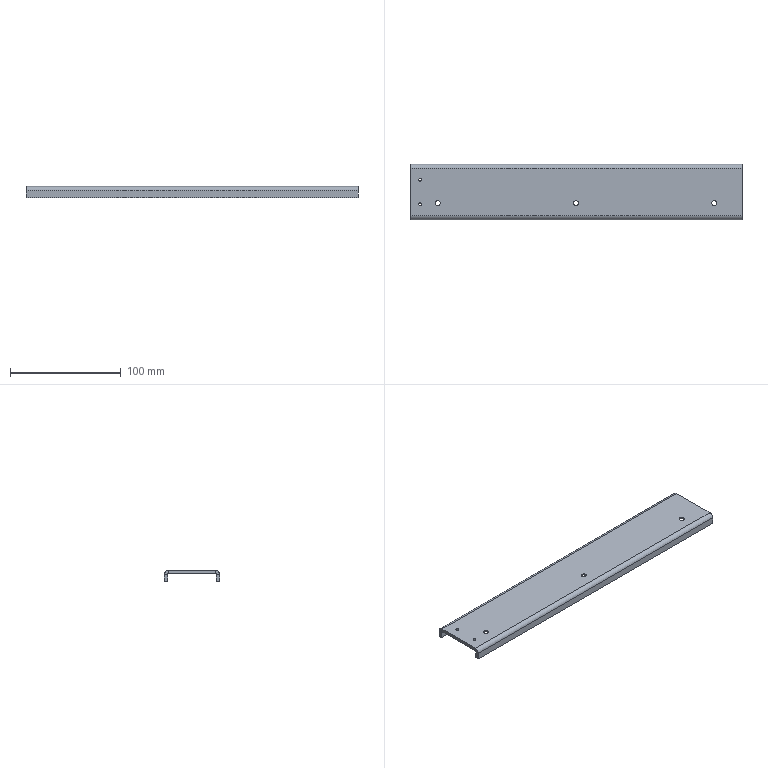Component | SolidWorks | SFTJ-04-DragChainSheet-Metal-1 | 1 solid | 38 faces | box 300 x 50 x 10 mm | volume 55526 mm3 | plane 18 | cylinder 14 | cone 6 | commonest cylinder face diameters 4.5 x6 2.5 x4 7.473 x2 1.473 x2 | material 201 Annealed Stainless Steel (SS)
STEP:
#1=COLOUR_RGB('',0.7922,0.8196,0.9333);
#2=FILL_AREA_STYLE_COLOUR('',#1);
#3=FILL_AREA_STYLE('',(#2));
#4=SURFACE_STYLE_FILL_AREA(#3);
#5=SURFACE_SIDE_STYLE('',(#4));
#6=SURFACE_STYLE_USAGE(.BOTH.,#5);
#7=PRESENTATION_STYLE_ASSIGNMENT((#6));
#8=CARTESIAN_POINT('',(-6.557,-0.5228,-1.827));
#9=VERTEX_POINT('',#8);
#10=CARTESIAN_POINT('',(-6.656,-0.5228,-1.827));
#11=VERTEX_POINT('',#10);
#12=CARTESIAN_POINT('',(-6.607,-0.5228,-1.827));
#13=DIRECTION('',(0.,-0.,-1.));
#14=DIRECTION('',(-1.,0.,0.));
#15=AXIS2_PLACEMENT_3D('',#12,#13,#14);
#16=CIRCLE('',#15,0.04921);
#17=EDGE_CURVE('',#9,#11,#16,.T.);
#18=ORIENTED_EDGE('',*,*,#17,.F.);
#19=CARTESIAN_POINT('',(-6.557,-0.5228,-1.945));
#20=VERTEX_POINT('',#19);
#21=CARTESIAN_POINT('',(-6.557,-0.5228,-1.945));
#22=DIRECTION('',(0.,-0.,-1.));
#23=VECTOR('',#22,39.37);
#24=LINE('',#21,#23);
#25=EDGE_CURVE('',#9,#20,#24,.T.);
#26=ORIENTED_EDGE('',*,*,#25,.T.);
#27=CARTESIAN_POINT('',(-6.656,-0.5228,-1.945));
#28=VERTEX_POINT('',#27);
#29=CARTESIAN_POINT('',(-6.607,-0.5228,-1.945));
#30=DIRECTION('',(0.,-0.,-1.));
#31=DIRECTION('',(-1.,0.,0.));
#32=AXIS2_PLACEMENT_3D('',#29,#30,#31);
#33=CIRCLE('',#32,0.04921);
#34=EDGE_CURVE('',#20,#28,#33,.T.);
#35=ORIENTED_EDGE('',*,*,#34,.T.);
#36=CARTESIAN_POINT('',(-6.656,-0.5228,-1.945));
#37=DIRECTION('',(0.,-0.,-1.));
#38=VECTOR('',#37,39.37);
#39=LINE('',#36,#38);
#40=EDGE_CURVE('',#11,#28,#39,.T.);
#41=ORIENTED_EDGE('',*,*,#40,.F.);
#42=EDGE_LOOP('',(#18,#26,#35,#41));
#43=FACE_OUTER_BOUND('',#42,.T.);
#44=CARTESIAN_POINT('',(-6.607,-0.5228,-1.945));
#45=DIRECTION('',(0.,-0.,-1.));
#46=DIRECTION('',(-1.,0.,0.));
#47=AXIS2_PLACEMENT_3D('',#44,#45,#46);
#48=CYLINDRICAL_SURFACE('',#47,0.04921);
#49=ADVANCED_FACE('',(#43),#48,.F.);
#50=CARTESIAN_POINT('',(-6.557,0.3433,-1.827));
#51=VERTEX_POINT('',#50);
#52=CARTESIAN_POINT('',(-6.656,0.3433,-1.827));
#53=VERTEX_POINT('',#52);
#54=CARTESIAN_POINT('',(-6.607,0.3433,-1.827));
#55=DIRECTION('',(0.,-0.,-1.));
#56=DIRECTION('',(-1.,0.,0.));
#57=AXIS2_PLACEMENT_3D('',#54,#55,#56);
#58=CIRCLE('',#57,0.04921);
#59=EDGE_CURVE('',#51,#53,#58,.T.);
#60=ORIENTED_EDGE('',*,*,#59,.F.);
#61=CARTESIAN_POINT('',(-6.557,0.3433,-1.945));
#62=VERTEX_POINT('',#61);
#63=CARTESIAN_POINT('',(-6.557,0.3433,-1.945));
#64=DIRECTION('',(0.,-0.,-1.));
#65=VECTOR('',#64,39.37);
#66=LINE('',#63,#65);
#67=EDGE_CURVE('',#51,#62,#66,.T.);
#68=ORIENTED_EDGE('',*,*,#67,.T.);
#69=CARTESIAN_POINT('',(-6.656,0.3433,-1.945));
#70=VERTEX_POINT('',#69);
#71=CARTESIAN_POINT('',(-6.607,0.3433,-1.945));
#72=DIRECTION('',(0.,-0.,-1.));
#73=DIRECTION('',(-1.,0.,0.));
#74=AXIS2_PLACEMENT_3D('',#71,#72,#73);
#75=CIRCLE('',#74,0.04921);
#76=EDGE_CURVE('',#62,#70,#75,.T.);
#77=ORIENTED_EDGE('',*,*,#76,.T.);
#78=CARTESIAN_POINT('',(-6.656,0.3433,-1.945));
#79=DIRECTION('',(0.,-0.,-1.));
#80=VECTOR('',#79,39.37);
#81=LINE('',#78,#80);
#82=EDGE_CURVE('',#53,#70,#81,.T.);
#83=ORIENTED_EDGE('',*,*,#82,.F.);
#84=EDGE_LOOP('',(#60,#68,#77,#83));
#85=FACE_OUTER_BOUND('',#84,.T.);
#86=CARTESIAN_POINT('',(-6.607,0.3433,-1.945));
#87=DIRECTION('',(0.,-0.,-1.));
#88=DIRECTION('',(-1.,0.,0.));
#89=AXIS2_PLACEMENT_3D('',#86,#87,#88);
#90=CYLINDRICAL_SURFACE('',#89,0.04921);
#91=ADVANCED_FACE('',(#85),#90,.F.);
#92=CARTESIAN_POINT('',(-5.896,-0.4834,-1.849));
#93=VERTEX_POINT('',#92);
#94=CARTESIAN_POINT('',(-6.073,-0.4834,-1.849));
#95=VERTEX_POINT('',#94);
#96=CARTESIAN_POINT('',(-5.985,-0.4834,-1.849));
#97=DIRECTION('',(0.,-0.,-1.));
#98=DIRECTION('',(-1.,0.,0.));
#99=AXIS2_PLACEMENT_3D('',#96,#97,#98);
#100=CIRCLE('',#99,0.08858);
#101=EDGE_CURVE('',#93,#95,#100,.T.);
#102=ORIENTED_EDGE('',*,*,#101,.F.);
#103=CARTESIAN_POINT('',(-5.8,-0.4834,-1.945));
#104=VERTEX_POINT('',#103);
#105=CARTESIAN_POINT('',(-5.8,-0.4834,-1.945));
#106=DIRECTION('',(0.7071,-0.,-0.7071));
#107=VECTOR('',#106,39.37);
#108=LINE('',#105,#107);
#109=EDGE_CURVE('',#93,#104,#108,.T.);
#110=ORIENTED_EDGE('',*,*,#109,.T.);
#111=CARTESIAN_POINT('',(-6.17,-0.4834,-1.945));
#112=VERTEX_POINT('',#111);
#113=CARTESIAN_POINT('',(-5.985,-0.4834,-1.945));
#114=DIRECTION('',(0.,-0.,-1.));
#115=DIRECTION('',(-1.,0.,0.));
#116=AXIS2_PLACEMENT_3D('',#113,#114,#115);
#117=CIRCLE('',#116,0.185);
#118=EDGE_CURVE('',#104,#112,#117,.T.);
#119=ORIENTED_EDGE('',*,*,#118,.T.);
#120=CARTESIAN_POINT('',(-6.17,-0.4834,-1.945));
#121=DIRECTION('',(-0.7071,-0.,-0.7071));
#122=VECTOR('',#121,39.37);
#123=LINE('',#120,#122);
#124=EDGE_CURVE('',#95,#112,#123,.T.);
#125=ORIENTED_EDGE('',*,*,#124,.F.);
#126=EDGE_LOOP('',(#102,#110,#119,#125));
#127=FACE_OUTER_BOUND('',#126,.T.);
#128=CARTESIAN_POINT('',(-5.985,-0.4834,-1.945));
#129=DIRECTION('',(0.,-0.,-1.));
#130=DIRECTION('',(-1.,0.,0.));
#131=AXIS2_PLACEMENT_3D('',#128,#129,#130);
#132=CONICAL_SURFACE('',#131,0.185,0.7854);
#133=ADVANCED_FACE('',(#127),#132,.F.);
#134=CARTESIAN_POINT('',(-5.896,-0.4834,-1.827));
#135=VERTEX_POINT('',#134);
#136=CARTESIAN_POINT('',(-6.073,-0.4834,-1.827));
#137=VERTEX_POINT('',#136);
#138=CARTESIAN_POINT('',(-5.985,-0.4834,-1.827));
#139=DIRECTION('',(0.,-0.,-1.));
#140=DIRECTION('',(-1.,0.,0.));
#141=AXIS2_PLACEMENT_3D('',#138,#139,#140);
#142=CIRCLE('',#141,0.08858);
#143=EDGE_CURVE('',#135,#137,#142,.T.);
#144=ORIENTED_EDGE('',*,*,#143,.F.);
#145=CARTESIAN_POINT('',(-5.896,-0.4834,-1.945));
#146=DIRECTION('',(0.,-0.,-1.));
#147=VECTOR('',#146,39.37);
#148=LINE('',#145,#147);
#149=EDGE_CURVE('',#135,#93,#148,.T.);
#150=ORIENTED_EDGE('',*,*,#149,.T.);
#151=ORIENTED_EDGE('',*,*,#101,.T.);
#152=CARTESIAN_POINT('',(-6.073,-0.4834,-1.945));
#153=DIRECTION('',(0.,-0.,-1.));
#154=VECTOR('',#153,39.37);
#155=LINE('',#152,#154);
#156=EDGE_CURVE('',#137,#95,#155,.T.);
#157=ORIENTED_EDGE('',*,*,#156,.F.);
#158=EDGE_LOOP('',(#144,#150,#151,#157));
#159=FACE_OUTER_BOUND('',#158,.T.);
#160=CARTESIAN_POINT('',(-5.985,-0.4834,-1.945));
#161=DIRECTION('',(0.,-0.,-1.));
#162=DIRECTION('',(-1.,0.,0.));
#163=AXIS2_PLACEMENT_3D('',#160,#161,#162);
#164=CYLINDRICAL_SURFACE('',#163,0.08858);
#165=ADVANCED_FACE('',(#159),#164,.F.);
#166=CARTESIAN_POINT('',(-0.9748,-0.4834,-1.849));
#167=VERTEX_POINT('',#166);
#168=CARTESIAN_POINT('',(-1.152,-0.4834,-1.849));
#169=VERTEX_POINT('',#168);
#170=CARTESIAN_POINT('',(-1.063,-0.4834,-1.849));
#171=DIRECTION('',(0.,-0.,-1.));
#172=DIRECTION('',(-1.,0.,0.));
#173=AXIS2_PLACEMENT_3D('',#170,#171,#172);
#174=CIRCLE('',#173,0.08858);
#175=EDGE_CURVE('',#167,#169,#174,.T.);
#176=ORIENTED_EDGE('',*,*,#175,.F.);
#177=CARTESIAN_POINT('',(-0.8783,-0.4834,-1.945));
#178=VERTEX_POINT('',#177);
#179=CARTESIAN_POINT('',(-0.8783,-0.4834,-1.945));
#180=DIRECTION('',(0.7071,-0.,-0.7071));
#181=VECTOR('',#180,39.37);
#182=LINE('',#179,#181);
#183=EDGE_CURVE('',#167,#178,#182,.T.);
#184=ORIENTED_EDGE('',*,*,#183,.T.);
#185=CARTESIAN_POINT('',(-1.248,-0.4834,-1.945));
#186=VERTEX_POINT('',#185);
#187=CARTESIAN_POINT('',(-1.063,-0.4834,-1.945));
#188=DIRECTION('',(0.,-0.,-1.));
#189=DIRECTION('',(-1.,0.,0.));
#190=AXIS2_PLACEMENT_3D('',#187,#188,#189);
#191=CIRCLE('',#190,0.185);
#192=EDGE_CURVE('',#178,#186,#191,.T.);
#193=ORIENTED_EDGE('',*,*,#192,.T.);
#194=CARTESIAN_POINT('',(-1.248,-0.4834,-1.945));
#195=DIRECTION('',(-0.7071,-0.,-0.7071));
#196=VECTOR('',#195,39.37);
#197=LINE('',#194,#196);
#198=EDGE_CURVE('',#169,#186,#197,.T.);
#199=ORIENTED_EDGE('',*,*,#198,.F.);
#200=EDGE_LOOP('',(#176,#184,#193,#199));
#201=FACE_OUTER_BOUND('',#200,.T.);
#202=CARTESIAN_POINT('',(-1.063,-0.4834,-1.945));
#203=DIRECTION('',(0.,-0.,-1.));
#204=DIRECTION('',(-1.,0.,0.));
#205=AXIS2_PLACEMENT_3D('',#202,#203,#204);
#206=CONICAL_SURFACE('',#205,0.185,0.7854);
#207=ADVANCED_FACE('',(#201),#206,.F.);
#208=CARTESIAN_POINT('',(-0.9748,-0.4834,-1.827));
#209=VERTEX_POINT('',#208);
#210=CARTESIAN_POINT('',(-1.152,-0.4834,-1.827));
#211=VERTEX_POINT('',#210);
#212=CARTESIAN_POINT('',(-1.063,-0.4834,-1.827));
#213=DIRECTION('',(0.,-0.,-1.));
#214=DIRECTION('',(-1.,0.,0.));
#215=AXIS2_PLACEMENT_3D('',#212,#213,#214);
#216=CIRCLE('',#215,0.08858);
#217=EDGE_CURVE('',#209,#211,#216,.T.);
#218=ORIENTED_EDGE('',*,*,#217,.F.);
#219=CARTESIAN_POINT('',(-0.9748,-0.4834,-1.945));
#220=DIRECTION('',(0.,-0.,-1.));
#221=VECTOR('',#220,39.37);
#222=LINE('',#219,#221);
#223=EDGE_CURVE('',#209,#167,#222,.T.);
#224=ORIENTED_EDGE('',*,*,#223,.T.);
#225=ORIENTED_EDGE('',*,*,#175,.T.);
#226=CARTESIAN_POINT('',(-1.152,-0.4834,-1.945));
#227=DIRECTION('',(0.,-0.,-1.));
#228=VECTOR('',#227,39.37);
#229=LINE('',#226,#228);
#230=EDGE_CURVE('',#211,#169,#229,.T.);
#231=ORIENTED_EDGE('',*,*,#230,.F.);
#232=EDGE_LOOP('',(#218,#224,#225,#231));
#233=FACE_OUTER_BOUND('',#232,.T.);
#234=CARTESIAN_POINT('',(-1.063,-0.4834,-1.945));
#235=DIRECTION('',(0.,-0.,-1.));
#236=DIRECTION('',(-1.,0.,0.));
#237=AXIS2_PLACEMENT_3D('',#234,#235,#236);
#238=CYLINDRICAL_SURFACE('',#237,0.08858);
#239=ADVANCED_FACE('',(#233),#238,.F.);
#240=CARTESIAN_POINT('',(3.946,-0.4834,-1.849));
#241=VERTEX_POINT('',#240);
#242=CARTESIAN_POINT('',(3.769,-0.4834,-1.849));
#243=VERTEX_POINT('',#242);
#244=CARTESIAN_POINT('',(3.858,-0.4834,-1.849));
#245=DIRECTION('',(0.,-0.,-1.));
#246=DIRECTION('',(-1.,0.,0.));
#247=AXIS2_PLACEMENT_3D('',#244,#245,#246);
#248=CIRCLE('',#247,0.08858);
#249=EDGE_CURVE('',#241,#243,#248,.T.);
#250=ORIENTED_EDGE('',*,*,#249,.F.);
#251=CARTESIAN_POINT('',(4.043,-0.4834,-1.945));
#252=VERTEX_POINT('',#251);
#253=CARTESIAN_POINT('',(4.043,-0.4834,-1.945));
#254=DIRECTION('',(0.7071,-0.,-0.7071));
#255=VECTOR('',#254,39.37);
#256=LINE('',#253,#255);
#257=EDGE_CURVE('',#241,#252,#256,.T.);
#258=ORIENTED_EDGE('',*,*,#257,.T.);
#259=CARTESIAN_POINT('',(3.673,-0.4834,-1.945));
#260=VERTEX_POINT('',#259);
#261=CARTESIAN_POINT('',(3.858,-0.4834,-1.945));
#262=DIRECTION('',(0.,-0.,-1.));
#263=DIRECTION('',(-1.,0.,0.));
#264=AXIS2_PLACEMENT_3D('',#261,#262,#263);
#265=CIRCLE('',#264,0.185);
#266=EDGE_CURVE('',#252,#260,#265,.T.);
#267=ORIENTED_EDGE('',*,*,#266,.T.);
#268=CARTESIAN_POINT('',(3.673,-0.4834,-1.945));
#269=DIRECTION('',(-0.7071,-0.,-0.7071));
#270=VECTOR('',#269,39.37);
#271=LINE('',#268,#270);
#272=EDGE_CURVE('',#243,#260,#271,.T.);
#273=ORIENTED_EDGE('',*,*,#272,.F.);
#274=EDGE_LOOP('',(#250,#258,#267,#273));
#275=FACE_OUTER_BOUND('',#274,.T.);
#276=CARTESIAN_POINT('',(3.858,-0.4834,-1.945));
#277=DIRECTION('',(0.,-0.,-1.));
#278=DIRECTION('',(-1.,0.,0.));
#279=AXIS2_PLACEMENT_3D('',#276,#277,#278);
#280=CONICAL_SURFACE('',#279,0.185,0.7854);
#281=ADVANCED_FACE('',(#275),#280,.F.);
#282=CARTESIAN_POINT('',(3.946,-0.4834,-1.827));
#283=VERTEX_POINT('',#282);
#284=CARTESIAN_POINT('',(3.769,-0.4834,-1.827));
#285=VERTEX_POINT('',#284);
#286=CARTESIAN_POINT('',(3.858,-0.4834,-1.827));
#287=DIRECTION('',(0.,-0.,-1.));
#288=DIRECTION('',(-1.,0.,0.));
#289=AXIS2_PLACEMENT_3D('',#286,#287,#288);
#290=CIRCLE('',#289,0.08858);
#291=EDGE_CURVE('',#283,#285,#290,.T.);
#292=ORIENTED_EDGE('',*,*,#291,.F.);
#293=CARTESIAN_POINT('',(3.946,-0.4834,-1.945));
#294=DIRECTION('',(0.,-0.,-1.));
#295=VECTOR('',#294,39.37);
#296=LINE('',#293,#295);
#297=EDGE_CURVE('',#283,#241,#296,.T.);
#298=ORIENTED_EDGE('',*,*,#297,.T.);
#299=ORIENTED_EDGE('',*,*,#249,.T.);
#300=CARTESIAN_POINT('',(3.769,-0.4834,-1.945));
#301=DIRECTION('',(0.,-0.,-1.));
#302=VECTOR('',#301,39.37);
#303=LINE('',#300,#302);
#304=EDGE_CURVE('',#285,#243,#303,.T.);
#305=ORIENTED_EDGE('',*,*,#304,.F.);
#306=EDGE_LOOP('',(#292,#298,#299,#305));
#307=FACE_OUTER_BOUND('',#306,.T.);
#308=CARTESIAN_POINT('',(3.858,-0.4834,-1.945));
#309=DIRECTION('',(0.,-0.,-1.));
#310=DIRECTION('',(-1.,0.,0.));
#311=AXIS2_PLACEMENT_3D('',#308,#309,#310);
#312=CYLINDRICAL_SURFACE('',#311,0.08858);
#313=ADVANCED_FACE('',(#307),#312,.F.);
#314=CARTESIAN_POINT('',(-6.969,0.7474,-1.827));
#315=VERTEX_POINT('',#314);
#316=CARTESIAN_POINT('',(-6.969,0.7474,-1.945));
#317=VERTEX_POINT('',#316);
#318=CARTESIAN_POINT('',(-6.969,0.7474,-1.827));
#319=DIRECTION('',(0.,-0.,-1.));
#320=VECTOR('',#319,39.37);
#321=LINE('',#318,#320);
#322=EDGE_CURVE('',#315,#317,#321,.T.);
#323=ORIENTED_EDGE('',*,*,#322,.F.);
#324=CARTESIAN_POINT('',(-6.969,0.8945,-1.974));
#325=VERTEX_POINT('',#324);
#326=CARTESIAN_POINT('',(-6.969,0.7474,-1.974));
#327=DIRECTION('',(1.,0.,0.));
#328=DIRECTION('',(0.,1.,0.));
#329=AXIS2_PLACEMENT_3D('',#326,#327,#328);
#330=CIRCLE('',#329,0.1471);
#331=EDGE_CURVE('',#325,#315,#330,.T.);
#332=ORIENTED_EDGE('',*,*,#331,.F.);
#333=CARTESIAN_POINT('',(-6.969,0.7764,-1.974));
#334=VERTEX_POINT('',#333);
#335=CARTESIAN_POINT('',(-6.969,0.7764,-1.974));
#336=DIRECTION('',(0.,1.,-0.));
#337=VECTOR('',#336,39.37);
#338=LINE('',#335,#337);
#339=EDGE_CURVE('',#334,#325,#338,.T.);
#340=ORIENTED_EDGE('',*,*,#339,.F.);
#341=CARTESIAN_POINT('',(-6.969,0.7474,-1.974));
#342=DIRECTION('',(1.,0.,0.));
#343=DIRECTION('',(0.,1.,0.));
#344=AXIS2_PLACEMENT_3D('',#341,#342,#343);
#345=CIRCLE('',#344,0.029);
#346=EDGE_CURVE('',#334,#317,#345,.T.);
#347=ORIENTED_EDGE('',*,*,#346,.T.);
#348=EDGE_LOOP('',(#323,#332,#340,#347));
#349=FACE_OUTER_BOUND('',#348,.T.);
#350=CARTESIAN_POINT('',(-6.969,0.7474,-1.827));
#351=DIRECTION('',(-1.,-0.,-0.));
#352=DIRECTION('',(0.,1.,-0.));
#353=AXIS2_PLACEMENT_3D('',#350,#351,#352);
#354=PLANE('',#353);
#355=ADVANCED_FACE('',(#349),#354,.T.);
#356=CARTESIAN_POINT('',(-6.969,-0.9269,-1.827));
#357=VERTEX_POINT('',#356);
#358=CARTESIAN_POINT('',(-6.969,-1.074,-1.827));
#359=DIRECTION('',(0.,-1.,0.));
#360=VECTOR('',#359,39.37);
#361=LINE('',#358,#360);
#362=EDGE_CURVE('',#315,#357,#361,.T.);
#363=ORIENTED_EDGE('',*,*,#362,.F.);
#364=ORIENTED_EDGE('',*,*,#322,.T.);
#365=CARTESIAN_POINT('',(-6.969,-0.9269,-1.945));
#366=VERTEX_POINT('',#365);
#367=CARTESIAN_POINT('',(-6.969,-1.074,-1.945));
#368=DIRECTION('',(0.,-1.,0.));
#369=VECTOR('',#368,39.37);
#370=LINE('',#367,#369);
#371=EDGE_CURVE('',#317,#366,#370,.T.);
#372=ORIENTED_EDGE('',*,*,#371,.T.);
#373=CARTESIAN_POINT('',(-6.969,-0.9269,-1.945));
#374=DIRECTION('',(-0.,0.,1.));
#375=VECTOR('',#374,39.37);
#376=LINE('',#373,#375);
#377=EDGE_CURVE('',#366,#357,#376,.T.);
#378=ORIENTED_EDGE('',*,*,#377,.T.);
#379=EDGE_LOOP('',(#363,#364,#372,#378));
#380=FACE_OUTER_BOUND('',#379,.T.);
#381=CARTESIAN_POINT('',(-6.969,0.7764,-1.974));
#382=DIRECTION('',(-1.,-0.,-0.));
#383=DIRECTION('',(0.,1.,-0.));
#384=AXIS2_PLACEMENT_3D('',#381,#382,#383);
#385=PLANE('',#384);
#386=ADVANCED_FACE('',(#380),#385,.T.);
#387=CARTESIAN_POINT('',(4.842,0.8945,-1.974));
#388=VERTEX_POINT('',#387);
#389=CARTESIAN_POINT('',(4.842,0.7764,-1.974));
#390=VERTEX_POINT('',#389);
#391=CARTESIAN_POINT('',(4.842,0.8945,-1.974));
#392=DIRECTION('',(0.,-1.,0.));
#393=VECTOR('',#392,39.37);
#394=LINE('',#391,#393);
#395=EDGE_CURVE('',#388,#390,#394,.T.);
#396=ORIENTED_EDGE('',*,*,#395,.F.);
#397=CARTESIAN_POINT('',(4.842,0.7474,-1.827));
#398=VERTEX_POINT('',#397);
#399=CARTESIAN_POINT('',(4.842,0.7474,-1.974));
#400=DIRECTION('',(1.,0.,0.));
#401=DIRECTION('',(0.,1.,0.));
#402=AXIS2_PLACEMENT_3D('',#399,#400,#401);
#403=CIRCLE('',#402,0.1471);
#404=EDGE_CURVE('',#388,#398,#403,.T.);
#405=ORIENTED_EDGE('',*,*,#404,.T.);
#406=CARTESIAN_POINT('',(4.842,0.7474,-1.945));
#407=VERTEX_POINT('',#406);
#408=CARTESIAN_POINT('',(4.842,0.7474,-1.945));
#409=DIRECTION('',(-0.,0.,1.));
#410=VECTOR('',#409,39.37);
#411=LINE('',#408,#410);
#412=EDGE_CURVE('',#407,#398,#411,.T.);
#413=ORIENTED_EDGE('',*,*,#412,.F.);
#414=CARTESIAN_POINT('',(4.842,0.7474,-1.974));
#415=DIRECTION('',(1.,0.,0.));
#416=DIRECTION('',(0.,1.,0.));
#417=AXIS2_PLACEMENT_3D('',#414,#415,#416);
#418=CIRCLE('',#417,0.029);
#419=EDGE_CURVE('',#390,#407,#418,.T.);
#420=ORIENTED_EDGE('',*,*,#419,.F.);
#421=EDGE_LOOP('',(#396,#405,#413,#420));
#422=FACE_OUTER_BOUND('',#421,.T.);
#423=CARTESIAN_POINT('',(4.842,0.8945,-1.974));
#424=DIRECTION('',(1.,0.,0.));
#425=DIRECTION('',(0.,-1.,0.));
#426=AXIS2_PLACEMENT_3D('',#423,#424,#425);
#427=PLANE('',#426);
#428=ADVANCED_FACE('',(#422),#427,.T.);
#429=CARTESIAN_POINT('',(4.842,0.8945,-2.221));
#430=VERTEX_POINT('',#429);
#431=CARTESIAN_POINT('',(4.842,0.8945,-1.827));
#432=DIRECTION('',(-0.,0.,1.));
#433=VECTOR('',#432,39.37);
#434=LINE('',#431,#433);
#435=EDGE_CURVE('',#430,#388,#434,.T.);
#436=ORIENTED_EDGE('',*,*,#435,.T.);
#437=ORIENTED_EDGE('',*,*,#395,.T.);
#438=CARTESIAN_POINT('',(4.842,0.7764,-2.221));
#439=VERTEX_POINT('',#438);
#440=CARTESIAN_POINT('',(4.842,0.7764,-1.827));
#441=DIRECTION('',(-0.,0.,1.));
#442=VECTOR('',#441,39.37);
#443=LINE('',#440,#442);
#444=EDGE_CURVE('',#439,#390,#443,.T.);
#445=ORIENTED_EDGE('',*,*,#444,.F.);
#446=CARTESIAN_POINT('',(4.842,0.7764,-2.221));
#447=DIRECTION('',(0.,1.,-0.));
#448=VECTOR('',#447,39.37);
#449=LINE('',#446,#448);
#450=EDGE_CURVE('',#439,#430,#449,.T.);
#451=ORIENTED_EDGE('',*,*,#450,.T.);
#452=EDGE_LOOP('',(#436,#437,#445,#451));
#453=FACE_OUTER_BOUND('',#452,.T.);
#454=CARTESIAN_POINT('',(4.842,0.7474,-1.945));
#455=DIRECTION('',(1.,0.,0.));
#456=DIRECTION('',(0.,-1.,0.));
#457=AXIS2_PLACEMENT_3D('',#454,#455,#456);
#458=PLANE('',#457);
#459=ADVANCED_FACE('',(#453),#458,.T.);
#460=CARTESIAN_POINT('',(-6.969,-1.074,-1.974));
#461=VERTEX_POINT('',#460);
#462=CARTESIAN_POINT('',(-6.969,-0.9559,-1.974));
#463=VERTEX_POINT('',#462);
#464=CARTESIAN_POINT('',(-6.969,-1.074,-1.974));
#465=DIRECTION('',(0.,1.,-0.));
#466=VECTOR('',#465,39.37);
#467=LINE('',#464,#466);
#468=EDGE_CURVE('',#461,#463,#467,.T.);
#469=ORIENTED_EDGE('',*,*,#468,.F.);
#470=CARTESIAN_POINT('',(-6.969,-0.9269,-1.974));
#471=DIRECTION('',(1.,0.,0.));
#472=DIRECTION('',(0.,1.,0.));
#473=AXIS2_PLACEMENT_3D('',#470,#471,#472);
#474=CIRCLE('',#473,0.1471);
#475=EDGE_CURVE('',#357,#461,#474,.T.);
#476=ORIENTED_EDGE('',*,*,#475,.F.);
#477=ORIENTED_EDGE('',*,*,#377,.F.);
#478=CARTESIAN_POINT('',(-6.969,-0.9269,-1.974));
#479=DIRECTION('',(1.,0.,0.));
#480=DIRECTION('',(0.,1.,0.));
#481=AXIS2_PLACEMENT_3D('',#478,#479,#480);
#482=CIRCLE('',#481,0.029);
#483=EDGE_CURVE('',#366,#463,#482,.T.);
#484=ORIENTED_EDGE('',*,*,#483,.T.);
#485=EDGE_LOOP('',(#469,#476,#477,#484));
#486=FACE_OUTER_BOUND('',#485,.T.);
#487=CARTESIAN_POINT('',(-6.969,-1.074,-1.974));
#488=DIRECTION('',(-1.,-0.,-0.));
#489=DIRECTION('',(0.,1.,-0.));
#490=AXIS2_PLACEMENT_3D('',#487,#488,#489);
#491=PLANE('',#490);
#492=ADVANCED_FACE('',(#486),#491,.T.);
#493=CARTESIAN_POINT('',(-6.969,-1.074,-2.221));
#494=VERTEX_POINT('',#493);
#495=CARTESIAN_POINT('',(-6.969,-1.074,-1.827));
#496=DIRECTION('',(0.,-0.,-1.));
#497=VECTOR('',#496,39.37);
#498=LINE('',#495,#497);
#499=EDGE_CURVE('',#461,#494,#498,.T.);
#500=ORIENTED_EDGE('',*,*,#499,.F.);
#501=ORIENTED_EDGE('',*,*,#468,.T.);
#502=CARTESIAN_POINT('',(-6.969,-0.9559,-2.221));
#503=VERTEX_POINT('',#502);
#504=CARTESIAN_POINT('',(-6.969,-0.9559,-1.827));
#505=DIRECTION('',(0.,-0.,-1.));
#506=VECTOR('',#505,39.37);
#507=LINE('',#504,#506);
#508=EDGE_CURVE('',#463,#503,#507,.T.);
#509=ORIENTED_EDGE('',*,*,#508,.T.);
#510=CARTESIAN_POINT('',(-6.969,-1.074,-2.221));
#511=DIRECTION('',(0.,1.,-0.));
#512=VECTOR('',#511,39.37);
#513=LINE('',#510,#512);
#514=EDGE_CURVE('',#494,#503,#513,.T.);
#515=ORIENTED_EDGE('',*,*,#514,.F.);
#516=EDGE_LOOP('',(#500,#501,#509,#515));
#517=FACE_OUTER_BOUND('',#516,.T.);
#518=CARTESIAN_POINT('',(-6.969,-0.9269,-1.945));
#519=DIRECTION('',(-1.,-0.,-0.));
#520=DIRECTION('',(0.,1.,-0.));
#521=AXIS2_PLACEMENT_3D('',#518,#519,#520);
#522=PLANE('',#521);
#523=ADVANCED_FACE('',(#517),#522,.T.);
#524=CARTESIAN_POINT('',(4.842,-0.9269,-1.827));
#525=VERTEX_POINT('',#524);
#526=CARTESIAN_POINT('',(4.842,-0.9269,-1.945));
#527=VERTEX_POINT('',#526);
#528=CARTESIAN_POINT('',(4.842,-0.9269,-1.827));
#529=DIRECTION('',(0.,-0.,-1.));
#530=VECTOR('',#529,39.37);
#531=LINE('',#528,#530);
#532=EDGE_CURVE('',#525,#527,#531,.T.);
#533=ORIENTED_EDGE('',*,*,#532,.F.);
#534=CARTESIAN_POINT('',(4.842,-1.074,-1.974));
#535=VERTEX_POINT('',#534);
#536=CARTESIAN_POINT('',(4.842,-0.9269,-1.974));
#537=DIRECTION('',(1.,0.,0.));
#538=DIRECTION('',(0.,1.,0.));
#539=AXIS2_PLACEMENT_3D('',#536,#537,#538);
#540=CIRCLE('',#539,0.1471);
#541=EDGE_CURVE('',#525,#535,#540,.T.);
#542=ORIENTED_EDGE('',*,*,#541,.T.);
#543=CARTESIAN_POINT('',(4.842,-0.9559,-1.974));
#544=VERTEX_POINT('',#543);
#545=CARTESIAN_POINT('',(4.842,-0.9559,-1.974));
#546=DIRECTION('',(0.,-1.,0.));
#547=VECTOR('',#546,39.37);
#548=LINE('',#545,#547);
#549=EDGE_CURVE('',#544,#535,#548,.T.);
#550=ORIENTED_EDGE('',*,*,#549,.F.);
#551=CARTESIAN_POINT('',(4.842,-0.9269,-1.974));
#552=DIRECTION('',(1.,0.,0.));
#553=DIRECTION('',(0.,1.,0.));
#554=AXIS2_PLACEMENT_3D('',#551,#552,#553);
#555=CIRCLE('',#554,0.029);
#556=EDGE_CURVE('',#527,#544,#555,.T.);
#557=ORIENTED_EDGE('',*,*,#556,.F.);
#558=EDGE_LOOP('',(#533,#542,#550,#557));
#559=FACE_OUTER_BOUND('',#558,.T.);
#560=CARTESIAN_POINT('',(4.842,-0.9269,-1.827));
#561=DIRECTION('',(1.,0.,0.));
#562=DIRECTION('',(0.,-1.,0.));
#563=AXIS2_PLACEMENT_3D('',#560,#561,#562);
#564=PLANE('',#563);
#565=ADVANCED_FACE('',(#559),#564,.T.);
#566=CARTESIAN_POINT('',(4.842,-1.074,-1.827));
#567=DIRECTION('',(0.,-1.,0.));
#568=VECTOR('',#567,39.37);
#569=LINE('',#566,#568);
#570=EDGE_CURVE('',#398,#525,#569,.T.);
#571=ORIENTED_EDGE('',*,*,#570,.T.);
#572=ORIENTED_EDGE('',*,*,#532,.T.);
#573=CARTESIAN_POINT('',(4.842,-1.074,-1.945));
#574=DIRECTION('',(0.,-1.,0.));
#575=VECTOR('',#574,39.37);
#576=LINE('',#573,#575);
#577=EDGE_CURVE('',#407,#527,#576,.T.);
#578=ORIENTED_EDGE('',*,*,#577,.F.);
#579=ORIENTED_EDGE('',*,*,#412,.T.);
#580=EDGE_LOOP('',(#571,#572,#578,#579));
#581=FACE_OUTER_BOUND('',#580,.T.);
#582=CARTESIAN_POINT('',(4.842,-0.9559,-1.974));
#583=DIRECTION('',(1.,0.,0.));
#584=DIRECTION('',(0.,-1.,0.));
#585=AXIS2_PLACEMENT_3D('',#582,#583,#584);
#586=PLANE('',#585);
#587=ADVANCED_FACE('',(#581),#586,.T.);
#588=CARTESIAN_POINT('',(4.842,-0.9559,-2.221));
#589=VERTEX_POINT('',#588);
#590=CARTESIAN_POINT('',(4.842,-0.9559,-1.827));
#591=DIRECTION('',(0.,-0.,-1.));
#592=VECTOR('',#591,39.37);
#593=LINE('',#590,#592);
#594=EDGE_CURVE('',#544,#589,#593,.T.);
#595=ORIENTED_EDGE('',*,*,#594,.T.);
#596=CARTESIAN_POINT('',(-6.969,-0.9559,-2.221));
#597=DIRECTION('',(1.,0.,0.));
#598=VECTOR('',#597,39.37);
#599=LINE('',#596,#598);
#600=EDGE_CURVE('',#503,#589,#599,.T.);
#601=ORIENTED_EDGE('',*,*,#600,.F.);
#602=ORIENTED_EDGE('',*,*,#508,.F.);
#603=CARTESIAN_POINT('',(-6.969,-0.9559,-1.974));
#604=DIRECTION('',(1.,0.,0.));
#605=VECTOR('',#604,39.37);
#606=LINE('',#603,#605);
#607=EDGE_CURVE('',#463,#544,#606,.T.);
#608=ORIENTED_EDGE('',*,*,#607,.T.);
#609=EDGE_LOOP('',(#595,#601,#602,#608));
#610=FACE_OUTER_BOUND('',#609,.T.);
#611=CARTESIAN_POINT('',(-6.969,-0.9559,-1.827));
#612=DIRECTION('',(-0.,-1.,0.));
#613=DIRECTION('',(-1.,0.,-0.));
#614=AXIS2_PLACEMENT_3D('',#611,#612,#613);
#615=PLANE('',#614);
#616=ADVANCED_FACE('',(#610),#615,.F.);
#617=CARTESIAN_POINT('',(4.842,-1.074,-2.221));
#618=VERTEX_POINT('',#617);
#619=CARTESIAN_POINT('',(4.842,-1.074,-2.221));
#620=DIRECTION('',(0.,1.,-0.));
#621=VECTOR('',#620,39.37);
#622=LINE('',#619,#621);
#623=EDGE_CURVE('',#618,#589,#622,.T.);
#624=ORIENTED_EDGE('',*,*,#623,.F.);
#625=CARTESIAN_POINT('',(-6.969,-1.074,-2.221));
#626=DIRECTION('',(1.,0.,0.));
#627=VECTOR('',#626,39.37);
#628=LINE('',#625,#627);
#629=EDGE_CURVE('',#494,#618,#628,.T.);
#630=ORIENTED_EDGE('',*,*,#629,.F.);
#631=ORIENTED_EDGE('',*,*,#514,.T.);
#632=ORIENTED_EDGE('',*,*,#600,.T.);
#633=EDGE_LOOP('',(#624,#630,#631,#632));
#634=FACE_OUTER_BOUND('',#633,.T.);
#635=CARTESIAN_POINT('',(-6.969,-1.074,-2.221));
#636=DIRECTION('',(0.,-0.,-1.));
#637=DIRECTION('',(-1.,0.,-0.));
#638=AXIS2_PLACEMENT_3D('',#635,#636,#637);
#639=PLANE('',#638);
#640=ADVANCED_FACE('',(#634),#639,.T.);
#641=CARTESIAN_POINT('',(4.842,-1.074,-1.827));
#642=DIRECTION('',(0.,-0.,-1.));
#643=VECTOR('',#642,39.37);
#644=LINE('',#641,#643);
#645=EDGE_CURVE('',#535,#618,#644,.T.);
#646=ORIENTED_EDGE('',*,*,#645,.F.);
#647=CARTESIAN_POINT('',(-6.969,-1.074,-1.974));
#648=DIRECTION('',(1.,0.,0.));
#649=VECTOR('',#648,39.37);
#650=LINE('',#647,#649);
#651=EDGE_CURVE('',#461,#535,#650,.T.);
#652=ORIENTED_EDGE('',*,*,#651,.F.);
#653=ORIENTED_EDGE('',*,*,#499,.T.);
#654=ORIENTED_EDGE('',*,*,#629,.T.);
#655=EDGE_LOOP('',(#646,#652,#653,#654));
#656=FACE_OUTER_BOUND('',#655,.T.);
#657=CARTESIAN_POINT('',(-6.969,-1.074,-1.827));
#658=DIRECTION('',(-0.,-1.,0.));
#659=DIRECTION('',(-1.,0.,-0.));
#660=AXIS2_PLACEMENT_3D('',#657,#658,#659);
#661=PLANE('',#660);
#662=ADVANCED_FACE('',(#656),#661,.T.);
#663=ORIENTED_EDGE('',*,*,#541,.F.);
#664=CARTESIAN_POINT('',(-6.969,-0.9269,-1.827));
#665=DIRECTION('',(1.,0.,0.));
#666=VECTOR('',#665,39.37);
#667=LINE('',#664,#666);
#668=EDGE_CURVE('',#357,#525,#667,.T.);
#669=ORIENTED_EDGE('',*,*,#668,.F.);
#670=ORIENTED_EDGE('',*,*,#475,.T.);
#671=ORIENTED_EDGE('',*,*,#651,.T.);
#672=EDGE_LOOP('',(#663,#669,#670,#671));
#673=FACE_OUTER_BOUND('',#672,.T.);
#674=CARTESIAN_POINT('',(-6.969,-0.9269,-1.974));
#675=DIRECTION('',(1.,0.,0.));
#676=DIRECTION('',(0.,-1.,0.));
#677=AXIS2_PLACEMENT_3D('',#674,#675,#676);
#678=CYLINDRICAL_SURFACE('',#677,0.1471);
#679=ADVANCED_FACE('',(#673),#678,.T.);
#680=CARTESIAN_POINT('',(-6.607,-0.5228,-1.827));
#681=DIRECTION('',(0.,-0.,-1.));
#682=DIRECTION('',(-1.,0.,0.));
#683=AXIS2_PLACEMENT_3D('',#680,#681,#682);
#684=CIRCLE('',#683,0.04921);
#685=EDGE_CURVE('',#11,#9,#684,.T.);
#686=ORIENTED_EDGE('',*,*,#685,.T.);
#687=ORIENTED_EDGE('',*,*,#17,.T.);
#688=EDGE_LOOP('',(#686,#687));
#689=FACE_BOUND('',#688,.T.);
#690=CARTESIAN_POINT('',(-6.607,0.3433,-1.827));
#691=DIRECTION('',(0.,-0.,-1.));
#692=DIRECTION('',(-1.,0.,0.));
#693=AXIS2_PLACEMENT_3D('',#690,#691,#692);
#694=CIRCLE('',#693,0.04921);
#695=EDGE_CURVE('',#53,#51,#694,.T.);
#696=ORIENTED_EDGE('',*,*,#695,.T.);
#697=ORIENTED_EDGE('',*,*,#59,.T.);
#698=EDGE_LOOP('',(#696,#697));
#699=FACE_BOUND('',#698,.T.);
#700=CARTESIAN_POINT('',(-5.985,-0.4834,-1.827));
#701=DIRECTION('',(0.,-0.,-1.));
#702=DIRECTION('',(-1.,0.,0.));
#703=AXIS2_PLACEMENT_3D('',#700,#701,#702);
#704=CIRCLE('',#703,0.08858);
#705=EDGE_CURVE('',#137,#135,#704,.T.);
#706=ORIENTED_EDGE('',*,*,#705,.T.);
#707=ORIENTED_EDGE('',*,*,#143,.T.);
#708=EDGE_LOOP('',(#706,#707));
#709=FACE_BOUND('',#708,.T.);
#710=CARTESIAN_POINT('',(-1.063,-0.4834,-1.827));
#711=DIRECTION('',(0.,-0.,-1.));
#712=DIRECTION('',(-1.,0.,0.));
#713=AXIS2_PLACEMENT_3D('',#710,#711,#712);
#714=CIRCLE('',#713,0.08858);
#715=EDGE_CURVE('',#211,#209,#714,.T.);
#716=ORIENTED_EDGE('',*,*,#715,.T.);
#717=ORIENTED_EDGE('',*,*,#217,.T.);
#718=EDGE_LOOP('',(#716,#717));
#719=FACE_BOUND('',#718,.T.);
#720=CARTESIAN_POINT('',(3.858,-0.4834,-1.827));
#721=DIRECTION('',(0.,-0.,-1.));
#722=DIRECTION('',(-1.,0.,0.));
#723=AXIS2_PLACEMENT_3D('',#720,#721,#722);
#724=CIRCLE('',#723,0.08858);
#725=EDGE_CURVE('',#285,#283,#724,.T.);
#726=ORIENTED_EDGE('',*,*,#725,.T.);
#727=ORIENTED_EDGE('',*,*,#291,.T.);
#728=EDGE_LOOP('',(#726,#727));
#729=FACE_BOUND('',#728,.T.);
#730=ORIENTED_EDGE('',*,*,#570,.F.);
#731=CARTESIAN_POINT('',(-6.969,0.7474,-1.827));
#732=DIRECTION('',(1.,0.,0.));
#733=VECTOR('',#732,39.37);
#734=LINE('',#731,#733);
#735=EDGE_CURVE('',#315,#398,#734,.T.);
#736=ORIENTED_EDGE('',*,*,#735,.F.);
#737=ORIENTED_EDGE('',*,*,#362,.T.);
#738=ORIENTED_EDGE('',*,*,#668,.T.);
#739=EDGE_LOOP('',(#730,#736,#737,#738));
#740=FACE_OUTER_BOUND('',#739,.T.);
#741=CARTESIAN_POINT('',(-6.969,-1.074,-1.827));
#742=DIRECTION('',(-0.,0.,1.));
#743=DIRECTION('',(1.,0.,0.));
#744=AXIS2_PLACEMENT_3D('',#741,#742,#743);
#745=PLANE('',#744);
#746=ADVANCED_FACE('',(#689,#699,#709,#719,#729,#740),#745,.T.);
#747=ORIENTED_EDGE('',*,*,#404,.F.);
#748=CARTESIAN_POINT('',(-6.969,0.8945,-1.974));
#749=DIRECTION('',(1.,0.,0.));
#750=VECTOR('',#749,39.37);
#751=LINE('',#748,#750);
#752=EDGE_CURVE('',#325,#388,#751,.T.);
#753=ORIENTED_EDGE('',*,*,#752,.F.);
#754=ORIENTED_EDGE('',*,*,#331,.T.);
#755=ORIENTED_EDGE('',*,*,#735,.T.);
#756=EDGE_LOOP('',(#747,#753,#754,#755));
#757=FACE_OUTER_BOUND('',#756,.T.);
#758=CARTESIAN_POINT('',(-6.969,0.7474,-1.974));
#759=DIRECTION('',(1.,0.,0.));
#760=DIRECTION('',(0.,-1.,0.));
#761=AXIS2_PLACEMENT_3D('',#758,#759,#760);
#762=CYLINDRICAL_SURFACE('',#761,0.1471);
#763=ADVANCED_FACE('',(#757),#762,.T.);
#764=ORIENTED_EDGE('',*,*,#435,.F.);
#765=CARTESIAN_POINT('',(-6.969,0.8945,-2.221));
#766=VERTEX_POINT('',#765);
#767=CARTESIAN_POINT('',(-6.969,0.8945,-2.221));
#768=DIRECTION('',(1.,0.,0.));
#769=VECTOR('',#768,39.37);
#770=LINE('',#767,#769);
#771=EDGE_CURVE('',#766,#430,#770,.T.);
#772=ORIENTED_EDGE('',*,*,#771,.F.);
#773=CARTESIAN_POINT('',(-6.969,0.8945,-1.827));
#774=DIRECTION('',(-0.,0.,1.));
#775=VECTOR('',#774,39.37);
#776=LINE('',#773,#775);
#777=EDGE_CURVE('',#766,#325,#776,.T.);
#778=ORIENTED_EDGE('',*,*,#777,.T.);
#779=ORIENTED_EDGE('',*,*,#752,.T.);
#780=EDGE_LOOP('',(#764,#772,#778,#779));
#781=FACE_OUTER_BOUND('',#780,.T.);
#782=CARTESIAN_POINT('',(-6.969,0.8945,-1.827));
#783=DIRECTION('',(0.,1.,-0.));
#784=DIRECTION('',(1.,0.,0.));
#785=AXIS2_PLACEMENT_3D('',#782,#783,#784);
#786=PLANE('',#785);
#787=ADVANCED_FACE('',(#781),#786,.T.);
#788=ORIENTED_EDGE('',*,*,#450,.F.);
#789=CARTESIAN_POINT('',(-6.969,0.7764,-2.221));
#790=VERTEX_POINT('',#789);
#791=CARTESIAN_POINT('',(-6.969,0.7764,-2.221));
#792=DIRECTION('',(1.,0.,0.));
#793=VECTOR('',#792,39.37);
#794=LINE('',#791,#793);
#795=EDGE_CURVE('',#790,#439,#794,.T.);
#796=ORIENTED_EDGE('',*,*,#795,.F.);
#797=CARTESIAN_POINT('',(-6.969,0.7764,-2.221));
#798=DIRECTION('',(0.,1.,-0.));
#799=VECTOR('',#798,39.37);
#800=LINE('',#797,#799);
#801=EDGE_CURVE('',#790,#766,#800,.T.);
#802=ORIENTED_EDGE('',*,*,#801,.T.);
#803=ORIENTED_EDGE('',*,*,#771,.T.);
#804=EDGE_LOOP('',(#788,#796,#802,#803));
#805=FACE_OUTER_BOUND('',#804,.T.);
#806=CARTESIAN_POINT('',(-6.969,0.7764,-2.221));
#807=DIRECTION('',(0.,-0.,-1.));
#808=DIRECTION('',(-1.,0.,-0.));
#809=AXIS2_PLACEMENT_3D('',#806,#807,#808);
#810=PLANE('',#809);
#811=ADVANCED_FACE('',(#805),#810,.T.);
#812=ORIENTED_EDGE('',*,*,#444,.T.);
#813=CARTESIAN_POINT('',(-6.969,0.7764,-1.974));
#814=DIRECTION('',(1.,0.,0.));
#815=VECTOR('',#814,39.37);
#816=LINE('',#813,#815);
#817=EDGE_CURVE('',#334,#390,#816,.T.);
#818=ORIENTED_EDGE('',*,*,#817,.F.);
#819=CARTESIAN_POINT('',(-6.969,0.7764,-1.827));
#820=DIRECTION('',(-0.,0.,1.));
#821=VECTOR('',#820,39.37);
#822=LINE('',#819,#821);
#823=EDGE_CURVE('',#790,#334,#822,.T.);
#824=ORIENTED_EDGE('',*,*,#823,.F.);
#825=ORIENTED_EDGE('',*,*,#795,.T.);
#826=EDGE_LOOP('',(#812,#818,#824,#825));
#827=FACE_OUTER_BOUND('',#826,.T.);
#828=CARTESIAN_POINT('',(-6.969,0.7764,-1.827));
#829=DIRECTION('',(0.,1.,-0.));
#830=DIRECTION('',(1.,0.,0.));
#831=AXIS2_PLACEMENT_3D('',#828,#829,#830);
#832=PLANE('',#831);
#833=ADVANCED_FACE('',(#827),#832,.F.);
#834=ORIENTED_EDGE('',*,*,#419,.T.);
#835=CARTESIAN_POINT('',(-6.969,0.7474,-1.945));
#836=DIRECTION('',(1.,0.,0.));
#837=VECTOR('',#836,39.37);
#838=LINE('',#835,#837);
#839=EDGE_CURVE('',#317,#407,#838,.T.);
#840=ORIENTED_EDGE('',*,*,#839,.F.);
#841=ORIENTED_EDGE('',*,*,#346,.F.);
#842=ORIENTED_EDGE('',*,*,#817,.T.);
#843=EDGE_LOOP('',(#834,#840,#841,#842));
#844=FACE_OUTER_BOUND('',#843,.T.);
#845=CARTESIAN_POINT('',(-6.969,0.7474,-1.974));
#846=DIRECTION('',(1.,0.,0.));
#847=DIRECTION('',(0.,-1.,0.));
#848=AXIS2_PLACEMENT_3D('',#845,#846,#847);
#849=CYLINDRICAL_SURFACE('',#848,0.029);
#850=ADVANCED_FACE('',(#844),#849,.F.);
#851=CARTESIAN_POINT('',(-6.607,-0.5228,-1.945));
#852=DIRECTION('',(0.,-0.,-1.));
#853=DIRECTION('',(-1.,0.,0.));
#854=AXIS2_PLACEMENT_3D('',#851,#852,#853);
#855=CIRCLE('',#854,0.04921);
#856=EDGE_CURVE('',#28,#20,#855,.T.);
#857=ORIENTED_EDGE('',*,*,#856,.F.);
#858=ORIENTED_EDGE('',*,*,#34,.F.);
#859=EDGE_LOOP('',(#857,#858));
#860=FACE_BOUND('',#859,.T.);
#861=CARTESIAN_POINT('',(-6.607,0.3433,-1.945));
#862=DIRECTION('',(0.,-0.,-1.));
#863=DIRECTION('',(-1.,0.,0.));
#864=AXIS2_PLACEMENT_3D('',#861,#862,#863);
#865=CIRCLE('',#864,0.04921);
#866=EDGE_CURVE('',#70,#62,#865,.T.);
#867=ORIENTED_EDGE('',*,*,#866,.F.);
#868=ORIENTED_EDGE('',*,*,#76,.F.);
#869=EDGE_LOOP('',(#867,#868));
#870=FACE_BOUND('',#869,.T.);
#871=CARTESIAN_POINT('',(-5.985,-0.4834,-1.945));
#872=DIRECTION('',(0.,-0.,-1.));
#873=DIRECTION('',(-1.,0.,0.));
#874=AXIS2_PLACEMENT_3D('',#871,#872,#873);
#875=CIRCLE('',#874,0.185);
#876=EDGE_CURVE('',#112,#104,#875,.T.);
#877=ORIENTED_EDGE('',*,*,#876,.F.);
#878=ORIENTED_EDGE('',*,*,#118,.F.);
#879=EDGE_LOOP('',(#877,#878));
#880=FACE_BOUND('',#879,.T.);
#881=CARTESIAN_POINT('',(-1.063,-0.4834,-1.945));
#882=DIRECTION('',(0.,-0.,-1.));
#883=DIRECTION('',(-1.,0.,0.));
#884=AXIS2_PLACEMENT_3D('',#881,#882,#883);
#885=CIRCLE('',#884,0.185);
#886=EDGE_CURVE('',#186,#178,#885,.T.);
#887=ORIENTED_EDGE('',*,*,#886,.F.);
#888=ORIENTED_EDGE('',*,*,#192,.F.);
#889=EDGE_LOOP('',(#887,#888));
#890=FACE_BOUND('',#889,.T.);
#891=CARTESIAN_POINT('',(3.858,-0.4834,-1.945));
#892=DIRECTION('',(0.,-0.,-1.));
#893=DIRECTION('',(-1.,0.,0.));
#894=AXIS2_PLACEMENT_3D('',#891,#892,#893);
#895=CIRCLE('',#894,0.185);
#896=EDGE_CURVE('',#260,#252,#895,.T.);
#897=ORIENTED_EDGE('',*,*,#896,.F.);
#898=ORIENTED_EDGE('',*,*,#266,.F.);
#899=EDGE_LOOP('',(#897,#898));
#900=FACE_BOUND('',#899,.T.);
#901=ORIENTED_EDGE('',*,*,#577,.T.);
#902=CARTESIAN_POINT('',(-6.969,-0.9269,-1.945));
#903=DIRECTION('',(1.,0.,0.));
#904=VECTOR('',#903,39.37);
#905=LINE('',#902,#904);
#906=EDGE_CURVE('',#366,#527,#905,.T.);
#907=ORIENTED_EDGE('',*,*,#906,.F.);
#908=ORIENTED_EDGE('',*,*,#371,.F.);
#909=ORIENTED_EDGE('',*,*,#839,.T.);
#910=EDGE_LOOP('',(#901,#907,#908,#909));
#911=FACE_OUTER_BOUND('',#910,.T.);
#912=CARTESIAN_POINT('',(-6.969,-1.074,-1.945));
#913=DIRECTION('',(-0.,0.,1.));
#914=DIRECTION('',(1.,0.,0.));
#915=AXIS2_PLACEMENT_3D('',#912,#913,#914);
#916=PLANE('',#915);
#917=ADVANCED_FACE('',(#860,#870,#880,#890,#900,#911),#916,.F.);
#918=ORIENTED_EDGE('',*,*,#556,.T.);
#919=ORIENTED_EDGE('',*,*,#607,.F.);
#920=ORIENTED_EDGE('',*,*,#483,.F.);
#921=ORIENTED_EDGE('',*,*,#906,.T.);
#922=EDGE_LOOP('',(#918,#919,#920,#921));
#923=FACE_OUTER_BOUND('',#922,.T.);
#924=CARTESIAN_POINT('',(-6.969,-0.9269,-1.974));
#925=DIRECTION('',(1.,0.,0.));
#926=DIRECTION('',(0.,-1.,0.));
#927=AXIS2_PLACEMENT_3D('',#924,#925,#926);
#928=CYLINDRICAL_SURFACE('',#927,0.029);
#929=ADVANCED_FACE('',(#923),#928,.F.);
#930=ORIENTED_EDGE('',*,*,#823,.T.);
#931=ORIENTED_EDGE('',*,*,#339,.T.);
#932=ORIENTED_EDGE('',*,*,#777,.F.);
#933=ORIENTED_EDGE('',*,*,#801,.F.);
#934=EDGE_LOOP('',(#930,#931,#932,#933));
#935=FACE_OUTER_BOUND('',#934,.T.);
#936=CARTESIAN_POINT('',(-6.969,-0.9269,-1.974));
#937=DIRECTION('',(-1.,-0.,-0.));
#938=DIRECTION('',(0.,1.,-0.));
#939=AXIS2_PLACEMENT_3D('',#936,#937,#938);
#940=PLANE('',#939);
#941=ADVANCED_FACE('',(#935),#940,.T.);
#942=ORIENTED_EDGE('',*,*,#594,.F.);
#943=ORIENTED_EDGE('',*,*,#549,.T.);
#944=ORIENTED_EDGE('',*,*,#645,.T.);
#945=ORIENTED_EDGE('',*,*,#623,.T.);
#946=EDGE_LOOP('',(#942,#943,#944,#945));
#947=FACE_OUTER_BOUND('',#946,.T.);
#948=CARTESIAN_POINT('',(4.842,-0.9269,-1.974));
#949=DIRECTION('',(-1.,-0.,-0.));
#950=DIRECTION('',(0.,1.,-0.));
#951=AXIS2_PLACEMENT_3D('',#948,#949,#950);
#952=PLANE('',#951);
#953=ADVANCED_FACE('',(#947),#952,.F.);
#954=ORIENTED_EDGE('',*,*,#297,.F.);
#955=ORIENTED_EDGE('',*,*,#725,.F.);
#956=ORIENTED_EDGE('',*,*,#304,.T.);
#957=CARTESIAN_POINT('',(3.858,-0.4834,-1.849));
#958=DIRECTION('',(0.,-0.,-1.));
#959=DIRECTION('',(-1.,0.,0.));
#960=AXIS2_PLACEMENT_3D('',#957,#958,#959);
#961=CIRCLE('',#960,0.08858);
#962=EDGE_CURVE('',#243,#241,#961,.T.);
#963=ORIENTED_EDGE('',*,*,#962,.T.);
#964=EDGE_LOOP('',(#954,#955,#956,#963));
#965=FACE_OUTER_BOUND('',#964,.T.);
#966=CARTESIAN_POINT('',(3.858,-0.4834,-1.945));
#967=DIRECTION('',(0.,-0.,-1.));
#968=DIRECTION('',(-1.,0.,0.));
#969=AXIS2_PLACEMENT_3D('',#966,#967,#968);
#970=CYLINDRICAL_SURFACE('',#969,0.08858);
#971=ADVANCED_FACE('',(#965),#970,.F.);
#972=ORIENTED_EDGE('',*,*,#257,.F.);
#973=ORIENTED_EDGE('',*,*,#962,.F.);
#974=ORIENTED_EDGE('',*,*,#272,.T.);
#975=ORIENTED_EDGE('',*,*,#896,.T.);
#976=EDGE_LOOP('',(#972,#973,#974,#975));
#977=FACE_OUTER_BOUND('',#976,.T.);
#978=CARTESIAN_POINT('',(3.858,-0.4834,-1.945));
#979=DIRECTION('',(0.,-0.,-1.));
#980=DIRECTION('',(-1.,0.,0.));
#981=AXIS2_PLACEMENT_3D('',#978,#979,#980);
#982=CONICAL_SURFACE('',#981,0.185,0.7854);
#983=ADVANCED_FACE('',(#977),#982,.F.);
#984=ORIENTED_EDGE('',*,*,#223,.F.);
#985=ORIENTED_EDGE('',*,*,#715,.F.);
#986=ORIENTED_EDGE('',*,*,#230,.T.);
#987=CARTESIAN_POINT('',(-1.063,-0.4834,-1.849));
#988=DIRECTION('',(0.,-0.,-1.));
#989=DIRECTION('',(-1.,0.,0.));
#990=AXIS2_PLACEMENT_3D('',#987,#988,#989);
#991=CIRCLE('',#990,0.08858);
#992=EDGE_CURVE('',#169,#167,#991,.T.);
#993=ORIENTED_EDGE('',*,*,#992,.T.);
#994=EDGE_LOOP('',(#984,#985,#986,#993));
#995=FACE_OUTER_BOUND('',#994,.T.);
#996=CARTESIAN_POINT('',(-1.063,-0.4834,-1.945));
#997=DIRECTION('',(0.,-0.,-1.));
#998=DIRECTION('',(-1.,0.,0.));
#999=AXIS2_PLACEMENT_3D('',#996,#997,#998);
#1000=CYLINDRICAL_SURFACE('',#999,0.08858);
#1001=ADVANCED_FACE('',(#995),#1000,.F.);
#1002=ORIENTED_EDGE('',*,*,#183,.F.);
#1003=ORIENTED_EDGE('',*,*,#992,.F.);
#1004=ORIENTED_EDGE('',*,*,#198,.T.);
#1005=ORIENTED_EDGE('',*,*,#886,.T.);
#1006=EDGE_LOOP('',(#1002,#1003,#1004,#1005));
#1007=FACE_OUTER_BOUND('',#1006,.T.);
#1008=CARTESIAN_POINT('',(-1.063,-0.4834,-1.945));
#1009=DIRECTION('',(0.,-0.,-1.));
#1010=DIRECTION('',(-1.,0.,0.));
#1011=AXIS2_PLACEMENT_3D('',#1008,#1009,#1010);
#1012=CONICAL_SURFACE('',#1011,0.185,0.7854);
#1013=ADVANCED_FACE('',(#1007),#1012,.F.);
#1014=ORIENTED_EDGE('',*,*,#149,.F.);
#1015=ORIENTED_EDGE('',*,*,#705,.F.);
#1016=ORIENTED_EDGE('',*,*,#156,.T.);
#1017=CARTESIAN_POINT('',(-5.985,-0.4834,-1.849));
#1018=DIRECTION('',(0.,-0.,-1.));
#1019=DIRECTION('',(-1.,0.,0.));
#1020=AXIS2_PLACEMENT_3D('',#1017,#1018,#1019);
#1021=CIRCLE('',#1020,0.08858);
#1022=EDGE_CURVE('',#95,#93,#1021,.T.);
#1023=ORIENTED_EDGE('',*,*,#1022,.T.);
#1024=EDGE_LOOP('',(#1014,#1015,#1016,#1023));
#1025=FACE_OUTER_BOUND('',#1024,.T.);
#1026=CARTESIAN_POINT('',(-5.985,-0.4834,-1.945));
#1027=DIRECTION('',(0.,-0.,-1.));
#1028=DIRECTION('',(-1.,0.,0.));
#1029=AXIS2_PLACEMENT_3D('',#1026,#1027,#1028);
#1030=CYLINDRICAL_SURFACE('',#1029,0.08858);
#1031=ADVANCED_FACE('',(#1025),#1030,.F.);
#1032=ORIENTED_EDGE('',*,*,#109,.F.);
#1033=ORIENTED_EDGE('',*,*,#1022,.F.);
#1034=ORIENTED_EDGE('',*,*,#124,.T.);
#1035=ORIENTED_EDGE('',*,*,#876,.T.);
#1036=EDGE_LOOP('',(#1032,#1033,#1034,#1035));
#1037=FACE_OUTER_BOUND('',#1036,.T.);
#1038=CARTESIAN_POINT('',(-5.985,-0.4834,-1.945));
#1039=DIRECTION('',(0.,-0.,-1.));
#1040=DIRECTION('',(-1.,0.,0.));
#1041=AXIS2_PLACEMENT_3D('',#1038,#1039,#1040);
#1042=CONICAL_SURFACE('',#1041,0.185,0.7854);
#1043=ADVANCED_FACE('',(#1037),#1042,.F.);
#1044=ORIENTED_EDGE('',*,*,#67,.F.);
#1045=ORIENTED_EDGE('',*,*,#695,.F.);
#1046=ORIENTED_EDGE('',*,*,#82,.T.);
#1047=ORIENTED_EDGE('',*,*,#866,.T.);
#1048=EDGE_LOOP('',(#1044,#1045,#1046,#1047));
#1049=FACE_OUTER_BOUND('',#1048,.T.);
#1050=CARTESIAN_POINT('',(-6.607,0.3433,-1.945));
#1051=DIRECTION('',(0.,-0.,-1.));
#1052=DIRECTION('',(-1.,0.,0.));
#1053=AXIS2_PLACEMENT_3D('',#1050,#1051,#1052);
#1054=CYLINDRICAL_SURFACE('',#1053,0.04921);
#1055=ADVANCED_FACE('',(#1049),#1054,.F.);
#1056=ORIENTED_EDGE('',*,*,#25,.F.);
#1057=ORIENTED_EDGE('',*,*,#685,.F.);
#1058=ORIENTED_EDGE('',*,*,#40,.T.);
#1059=ORIENTED_EDGE('',*,*,#856,.T.);
#1060=EDGE_LOOP('',(#1056,#1057,#1058,#1059));
#1061=FACE_OUTER_BOUND('',#1060,.T.);
#1062=CARTESIAN_POINT('',(-6.607,-0.5228,-1.945));
#1063=DIRECTION('',(0.,-0.,-1.));
#1064=DIRECTION('',(-1.,0.,0.));
#1065=AXIS2_PLACEMENT_3D('',#1062,#1063,#1064);
#1066=CYLINDRICAL_SURFACE('',#1065,0.04921);
#1067=ADVANCED_FACE('',(#1061),#1066,.F.);
#1068=CLOSED_SHELL('',(#49,#91,#133,#165,#207,#239,#281,#313,#355,#386,#428,#459,#492,#523,#565,#587,#616,#640,#662,#679,#746,#763,#787,#811,#833,#850,#917,#929,#941,#953,#971,#983,#1001,#1013,#1031,#1043,#1055,#1067));
#1069=MANIFOLD_SOLID_BREP('',#1068);
#1070=STYLED_ITEM('',(#7),#1069);
#1071=PRESENTATION_LAYER_ASSIGNMENT('','',(#1070));
#1072=CARTESIAN_POINT('',(0.,0.,0.));
#1073=DIRECTION('',(0.,0.,1.));
#1074=DIRECTION('',(1.,0.,0.));
#1075=AXIS2_PLACEMENT_3D('',#1072,#1073,#1074);
#1076=(LENGTH_UNIT()NAMED_UNIT(*)SI_UNIT($,.METRE.));
#1077=LENGTH_MEASURE_WITH_UNIT(LENGTH_MEASURE(0.0254),#1076);
#1078=DIMENSIONAL_EXPONENTS(1.,0.,0.,0.,0.,0.,0.);
#1079=(CONVERSION_BASED_UNIT('',#1077)LENGTH_UNIT()NAMED_UNIT(#1078));
#1080=UNCERTAINTY_MEASURE_WITH_UNIT(LENGTH_MEASURE(0.00001),#1079,'','');
#1081=(NAMED_UNIT(*)PLANE_ANGLE_UNIT()SI_UNIT($,.RADIAN.));
#1082=(NAMED_UNIT(*)SI_UNIT($,.STERADIAN.)SOLID_ANGLE_UNIT());
#1083=(GEOMETRIC_REPRESENTATION_CONTEXT(3)GLOBAL_UNCERTAINTY_ASSIGNED_CONTEXT((#1080))GLOBAL_UNIT_ASSIGNED_CONTEXT((#1079,#1081,#1082))REPRESENTATION_CONTEXT('',''));
#1084=ADVANCED_BREP_SHAPE_REPRESENTATION('',(#1069,#1075),#1083);
#1085=(LENGTH_UNIT()NAMED_UNIT(*)SI_UNIT($,.METRE.));
#1086=LENGTH_MEASURE_WITH_UNIT(LENGTH_MEASURE(0.0254),#1085);
#1087=DIMENSIONAL_EXPONENTS(1.,0.,0.,0.,0.,0.,0.);
#1088=(CONVERSION_BASED_UNIT('',#1086)LENGTH_UNIT()NAMED_UNIT(#1087));
#1089=UNCERTAINTY_MEASURE_WITH_UNIT(LENGTH_MEASURE(0.00001),#1088,'','');
#1090=(NAMED_UNIT(*)PLANE_ANGLE_UNIT()SI_UNIT($,.RADIAN.));
#1091=(NAMED_UNIT(*)SI_UNIT($,.STERADIAN.)SOLID_ANGLE_UNIT());
#1092=(GEOMETRIC_REPRESENTATION_CONTEXT(3)GLOBAL_UNCERTAINTY_ASSIGNED_CONTEXT((#1089))GLOBAL_UNIT_ASSIGNED_CONTEXT((#1088,#1090,#1091))REPRESENTATION_CONTEXT('',''));
#1093=MECHANICAL_DESIGN_GEOMETRIC_PRESENTATION_REPRESENTATION('',(#1070),#1092);